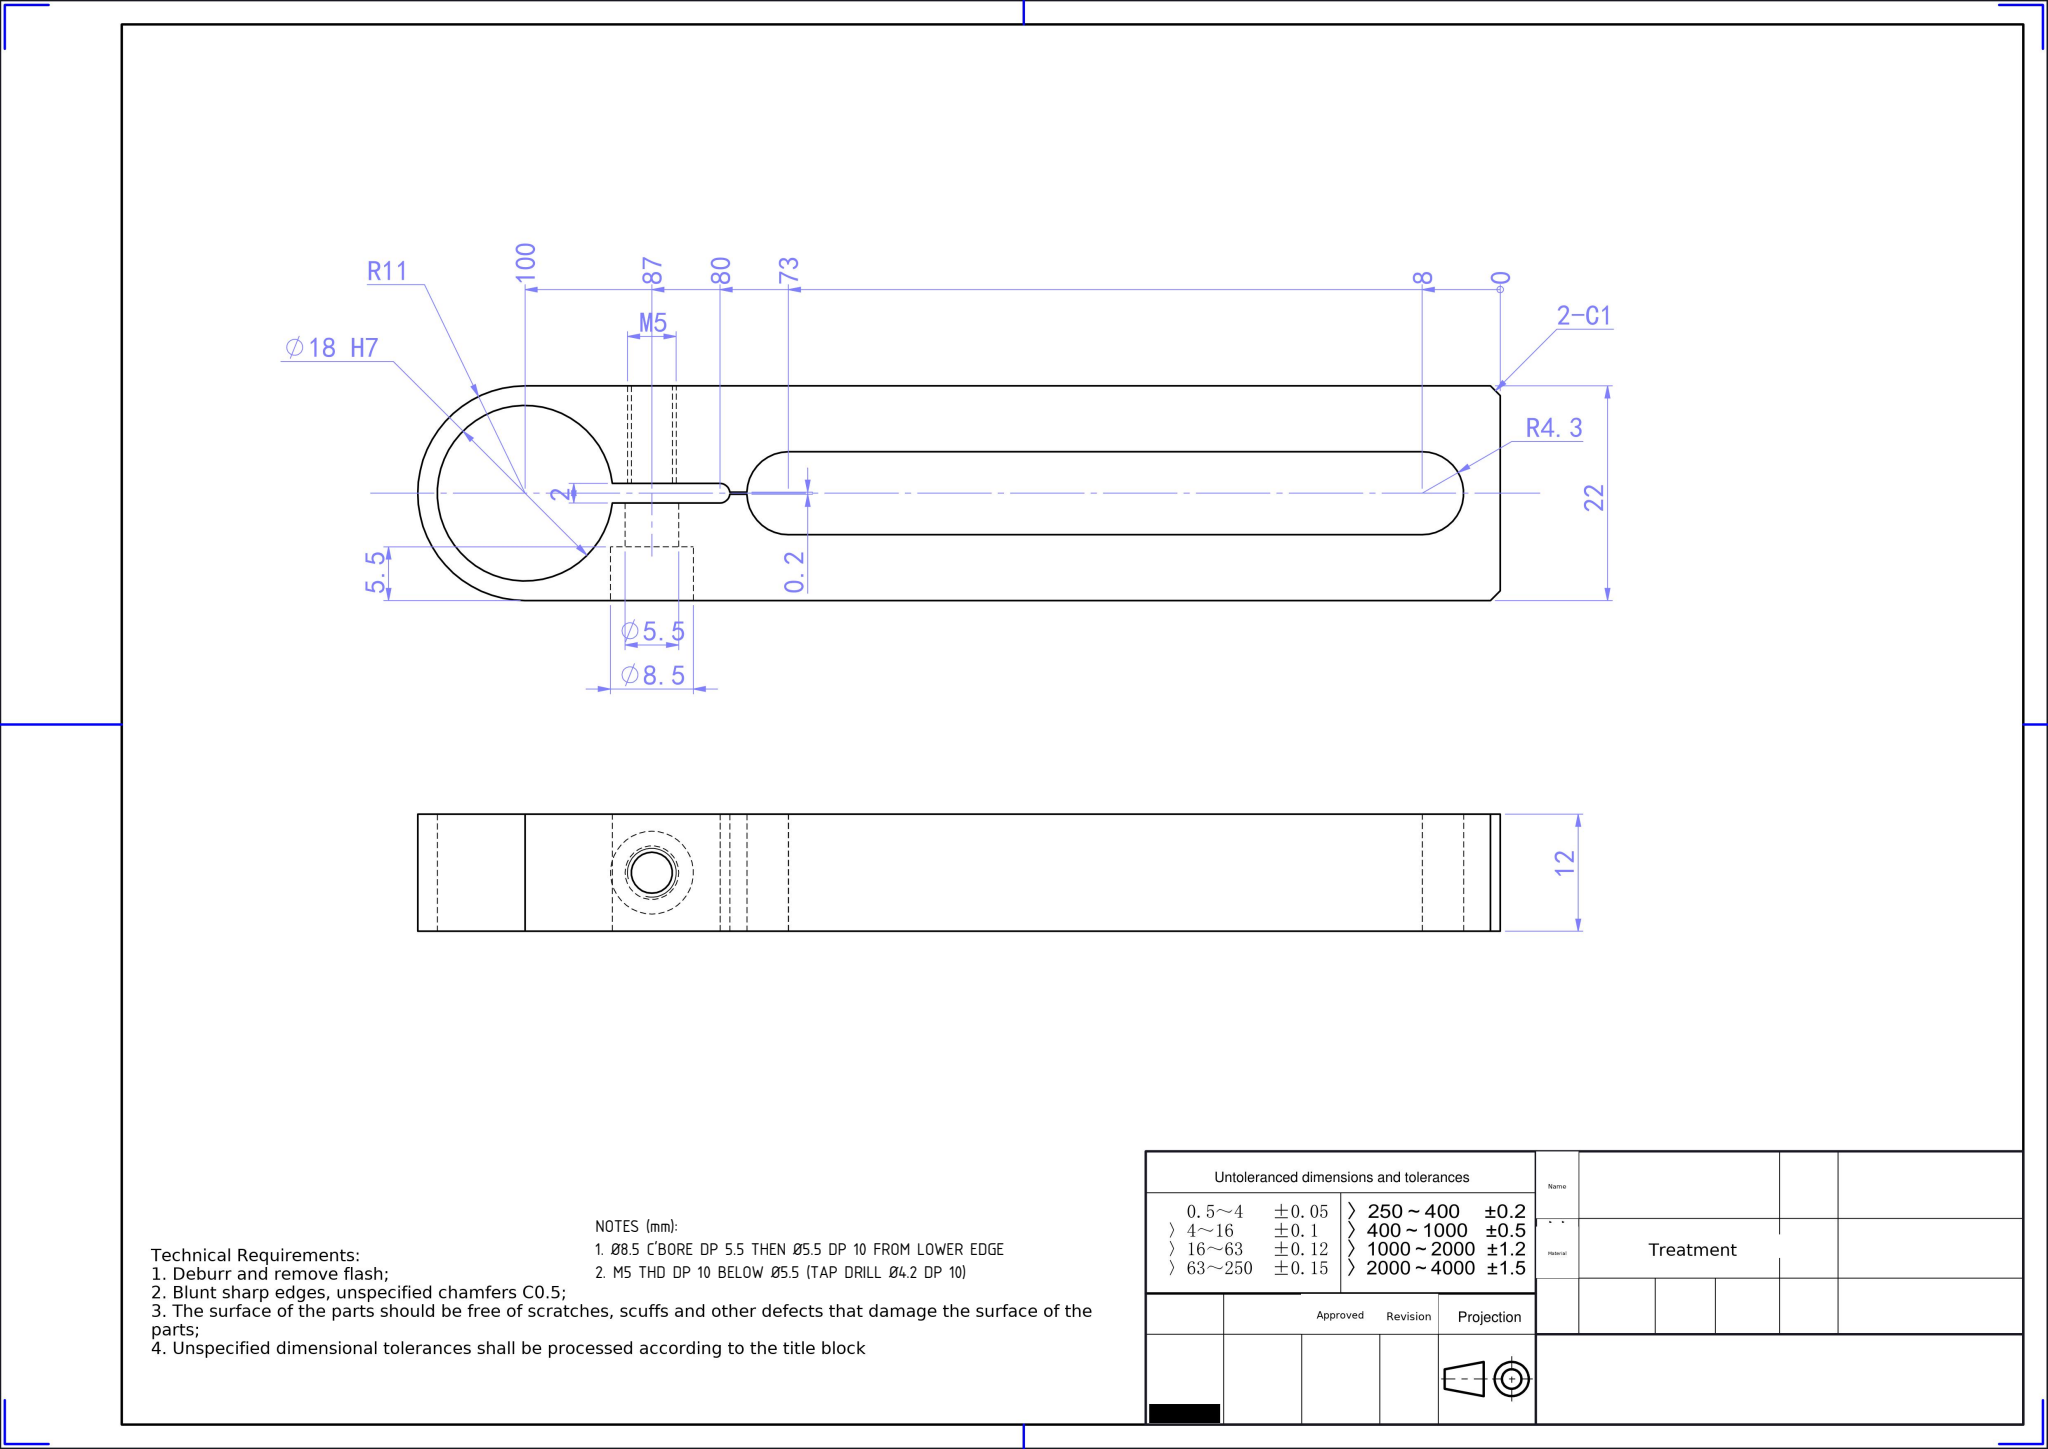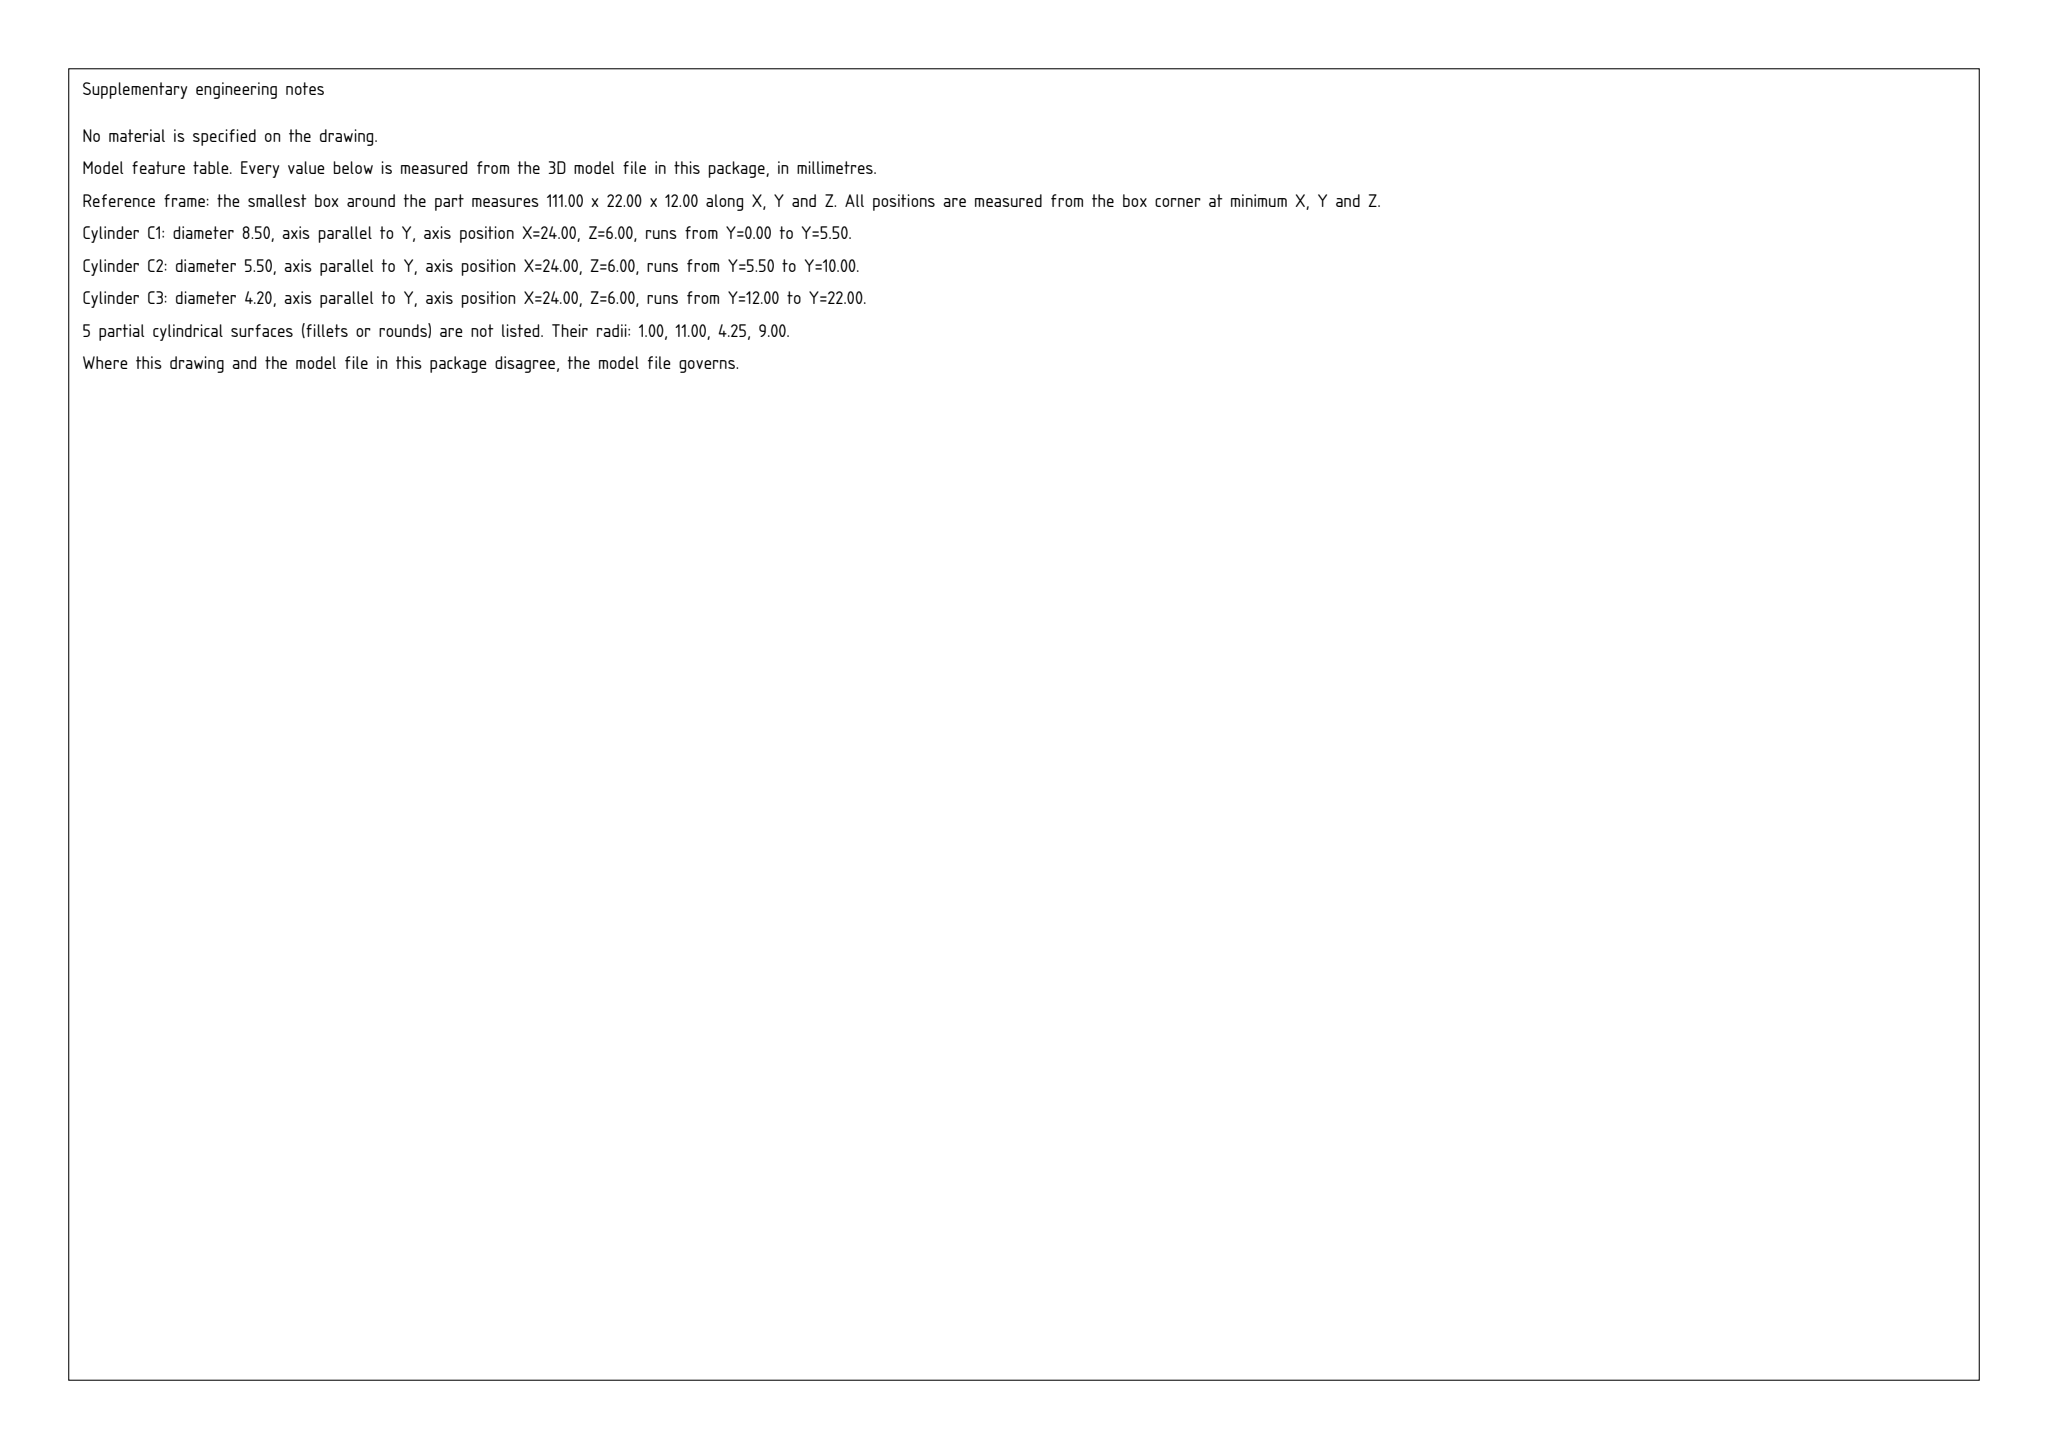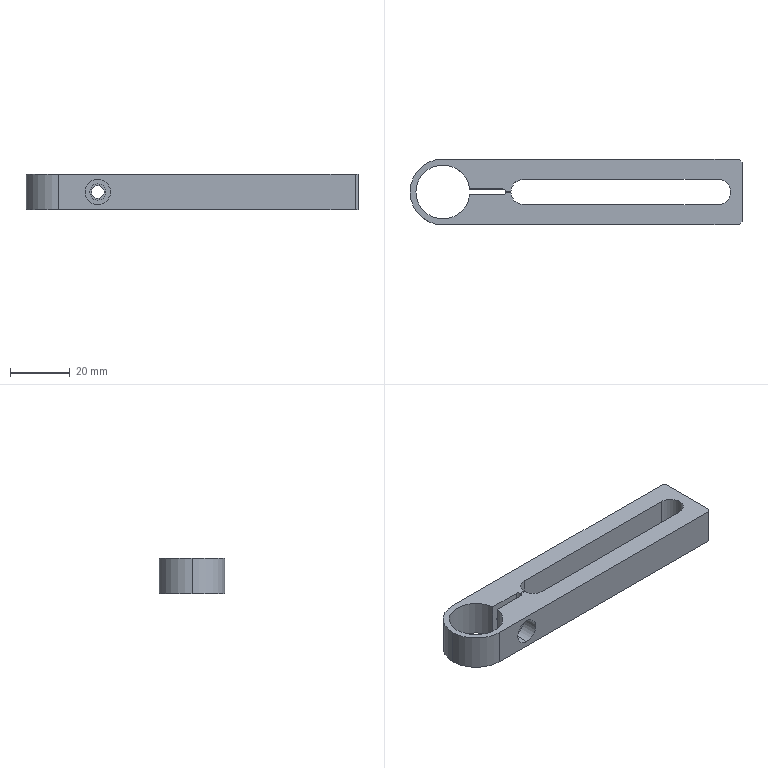Part | SolidWorks | mm | 1 solid | 29 faces | box 111 x 22 x 12 mm | volume 17459 mm3 | cylinder 15 | plane 14 | commonest cylinder face diameters 8.5 x5 5.5 x2 4.2 x2 18 x2 22 x2 2 x2
Drawing notes:
Ø8.5 C'BORE DP 5.5 THEN Ø5.5 DP 10 FROM LOWER EDGE | from the solid: Y-axis cyls at x=24,z=6: Ø8.5 L=5.5 (y 0-5.5), Ø5.5 L=4.5 (y 5.5-10)
M5 THD DP 10 BELOW Ø5.5 (TAP DRILL Ø4.2 DP 10) | from the solid: Y-axis cyl Ø4.2 L=10 at x=24,z=6, starting at y=10 plane